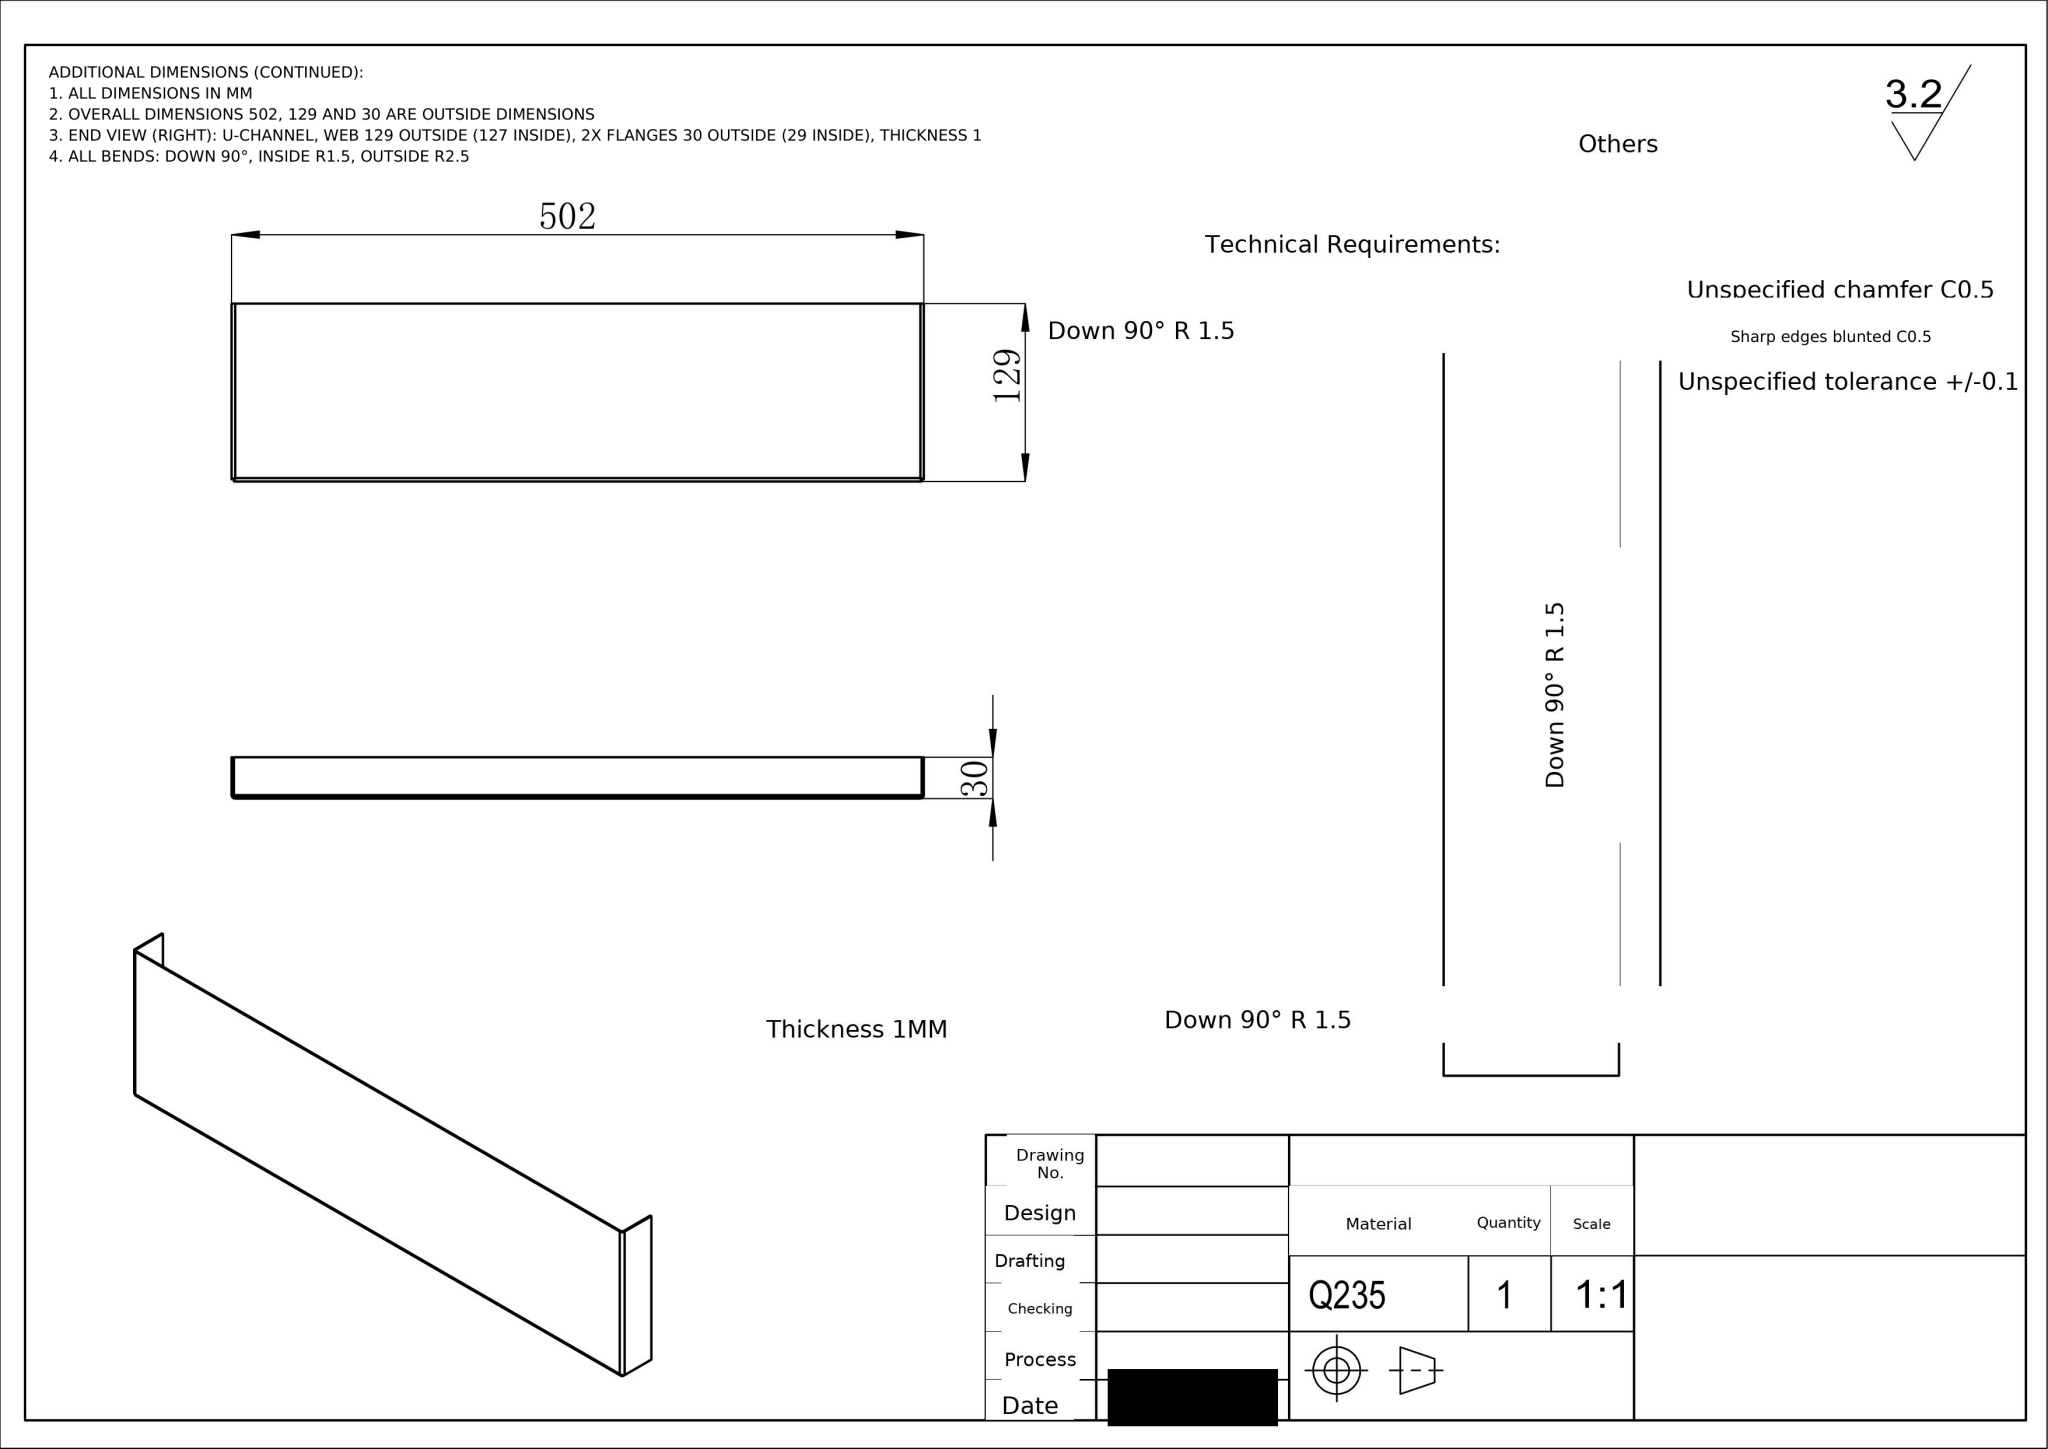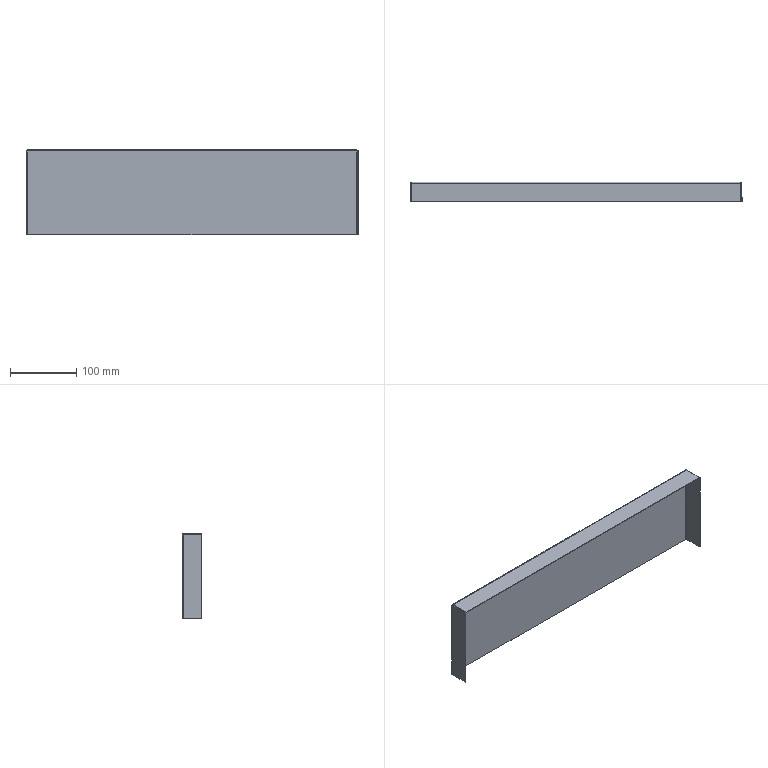Part | NX | mm | 1 solid | 30 faces | box 502 x 30 x 129 mm | volume 85944 mm3 | plane 20 | cylinder 6 | spline 4 | commonest cylinder face diameters 5 x3 3 x3